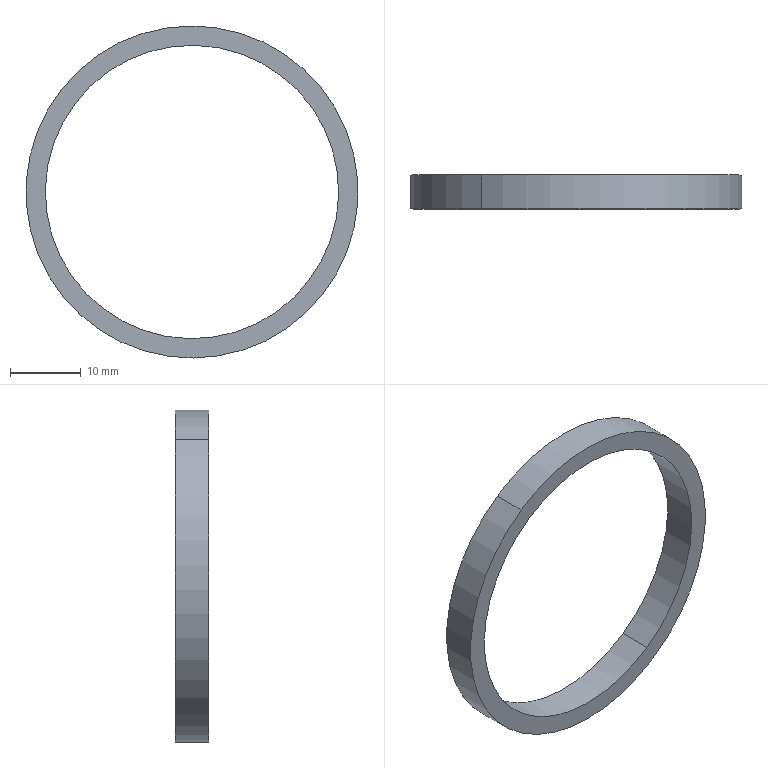Component | SolidWorks | 15-1 | 1 solid | 6 faces | box 47 x 4.8 x 47 mm | volume 1829 mm3 | cylinder 4 | plane 2 | commonest cylinder face diameters 41.52 x2 47 x2
build123d program:
from build123d import *

# Parameters (mm, degrees)
SKETCH1_R           = 23.5
SKETCH1_R_2         = 20.76
BOSS_EXTRUDE1_DEPTH = 4.8


with BuildPart() as part:
    # Sketch1 → Boss-Extrude1 (new body)
    with BuildSketch(Plane(origin=(0, 0, 0), x_dir=(1, 0, 0), z_dir=(0, 1, 0))):
        with Locations(Location((0, 0, 0), (0, 0, 270))):
            Circle(SKETCH1_R)
        with Locations(Location((0, 0, 0), (0, 0, 270))):
            Circle(SKETCH1_R_2, mode=Mode.SUBTRACT)
    extrude(amount=BOSS_EXTRUDE1_DEPTH)


solid = part.part

# Placed as in the assembly
solid = solid.moved(Location((0, -58.1, 0), (0, 0, 0)))
STEP:
#1=COLOUR_RGB('',0.7922,0.8196,0.9333);
#2=FILL_AREA_STYLE_COLOUR('',#1);
#3=FILL_AREA_STYLE('',(#2));
#4=SURFACE_STYLE_FILL_AREA(#3);
#5=SURFACE_SIDE_STYLE('',(#4));
#6=SURFACE_STYLE_USAGE(.BOTH.,#5);
#7=PRESENTATION_STYLE_ASSIGNMENT((#6));
#8=CARTESIAN_POINT('',(0.465,-2.098,-0.6722));
#9=VERTEX_POINT('',#8);
#10=CARTESIAN_POINT('',(-0.465,-2.098,0.6722));
#11=VERTEX_POINT('',#10);
#12=CARTESIAN_POINT('',(0.,-2.098,0.));
#13=DIRECTION('',(0.,1.,0.));
#14=DIRECTION('',(-0.5689,0.,0.8224));
#15=AXIS2_PLACEMENT_3D('',#12,#13,#14);
#16=CIRCLE('',#15,0.8173);
#17=EDGE_CURVE('',#9,#11,#16,.T.);
#18=ORIENTED_EDGE('',*,*,#17,.T.);
#19=CARTESIAN_POINT('',(-0.465,-2.287,0.6722));
#20=VERTEX_POINT('',#19);
#21=CARTESIAN_POINT('',(-0.465,-2.098,0.6722));
#22=DIRECTION('',(0.,-1.,0.));
#23=VECTOR('',#22,39.37);
#24=LINE('',#21,#23);
#25=EDGE_CURVE('',#11,#20,#24,.T.);
#26=ORIENTED_EDGE('',*,*,#25,.T.);
#27=CARTESIAN_POINT('',(0.465,-2.287,-0.6722));
#28=VERTEX_POINT('',#27);
#29=CARTESIAN_POINT('',(0.,-2.287,0.));
#30=DIRECTION('',(0.,1.,0.));
#31=DIRECTION('',(-0.5689,0.,0.8224));
#32=AXIS2_PLACEMENT_3D('',#29,#30,#31);
#33=CIRCLE('',#32,0.8173);
#34=EDGE_CURVE('',#28,#20,#33,.T.);
#35=ORIENTED_EDGE('',*,*,#34,.F.);
#36=CARTESIAN_POINT('',(0.465,-2.098,-0.6722));
#37=DIRECTION('',(0.,-1.,0.));
#38=VECTOR('',#37,39.37);
#39=LINE('',#36,#38);
#40=EDGE_CURVE('',#9,#28,#39,.T.);
#41=ORIENTED_EDGE('',*,*,#40,.F.);
#42=EDGE_LOOP('',(#18,#26,#35,#41));
#43=FACE_OUTER_BOUND('',#42,.T.);
#44=CARTESIAN_POINT('',(0.,-2.098,0.));
#45=DIRECTION('',(0.,-1.,0.));
#46=DIRECTION('',(0.5689,0.,-0.8224));
#47=AXIS2_PLACEMENT_3D('',#44,#45,#46);
#48=CYLINDRICAL_SURFACE('',#47,0.8173);
#49=ADVANCED_FACE('',(#43),#48,.F.);
#50=CARTESIAN_POINT('',(-0.5264,-2.098,0.7609));
#51=VERTEX_POINT('',#50);
#52=CARTESIAN_POINT('',(0.5264,-2.098,-0.7609));
#53=VERTEX_POINT('',#52);
#54=CARTESIAN_POINT('',(0.,-2.098,0.));
#55=DIRECTION('',(0.,1.,0.));
#56=DIRECTION('',(-0.5689,0.,0.8224));
#57=AXIS2_PLACEMENT_3D('',#54,#55,#56);
#58=CIRCLE('',#57,0.9252);
#59=EDGE_CURVE('',#51,#53,#58,.T.);
#60=ORIENTED_EDGE('',*,*,#59,.F.);
#61=CARTESIAN_POINT('',(-0.5264,-2.287,0.7609));
#62=VERTEX_POINT('',#61);
#63=CARTESIAN_POINT('',(-0.5264,-2.098,0.7609));
#64=DIRECTION('',(0.,-1.,0.));
#65=VECTOR('',#64,39.37);
#66=LINE('',#63,#65);
#67=EDGE_CURVE('',#51,#62,#66,.T.);
#68=ORIENTED_EDGE('',*,*,#67,.T.);
#69=CARTESIAN_POINT('',(0.5264,-2.287,-0.7609));
#70=VERTEX_POINT('',#69);
#71=CARTESIAN_POINT('',(0.,-2.287,0.));
#72=DIRECTION('',(0.,1.,0.));
#73=DIRECTION('',(-0.5689,0.,0.8224));
#74=AXIS2_PLACEMENT_3D('',#71,#72,#73);
#75=CIRCLE('',#74,0.9252);
#76=EDGE_CURVE('',#62,#70,#75,.T.);
#77=ORIENTED_EDGE('',*,*,#76,.T.);
#78=CARTESIAN_POINT('',(0.5264,-2.098,-0.7609));
#79=DIRECTION('',(0.,-1.,0.));
#80=VECTOR('',#79,39.37);
#81=LINE('',#78,#80);
#82=EDGE_CURVE('',#53,#70,#81,.T.);
#83=ORIENTED_EDGE('',*,*,#82,.F.);
#84=EDGE_LOOP('',(#60,#68,#77,#83));
#85=FACE_OUTER_BOUND('',#84,.T.);
#86=CARTESIAN_POINT('',(0.,-2.098,0.));
#87=DIRECTION('',(0.,-1.,0.));
#88=DIRECTION('',(0.5689,0.,-0.8224));
#89=AXIS2_PLACEMENT_3D('',#86,#87,#88);
#90=CYLINDRICAL_SURFACE('',#89,0.9252);
#91=ADVANCED_FACE('',(#85),#90,.T.);
#92=CARTESIAN_POINT('',(0.,-2.098,0.));
#93=DIRECTION('',(0.,1.,0.));
#94=DIRECTION('',(-0.5689,0.,0.8224));
#95=AXIS2_PLACEMENT_3D('',#92,#93,#94);
#96=CIRCLE('',#95,0.9252);
#97=EDGE_CURVE('',#53,#51,#96,.T.);
#98=ORIENTED_EDGE('',*,*,#97,.T.);
#99=ORIENTED_EDGE('',*,*,#59,.T.);
#100=EDGE_LOOP('',(#98,#99));
#101=FACE_OUTER_BOUND('',#100,.T.);
#102=ORIENTED_EDGE('',*,*,#17,.F.);
#103=CARTESIAN_POINT('',(0.,-2.098,0.));
#104=DIRECTION('',(0.,1.,0.));
#105=DIRECTION('',(-0.5689,0.,0.8224));
#106=AXIS2_PLACEMENT_3D('',#103,#104,#105);
#107=CIRCLE('',#106,0.8173);
#108=EDGE_CURVE('',#11,#9,#107,.T.);
#109=ORIENTED_EDGE('',*,*,#108,.F.);
#110=EDGE_LOOP('',(#102,#109));
#111=FACE_BOUND('',#110,.T.);
#112=CARTESIAN_POINT('',(0.,-2.098,0.));
#113=DIRECTION('',(0.,1.,0.));
#114=DIRECTION('',(-0.5689,0.,0.8224));
#115=AXIS2_PLACEMENT_3D('',#112,#113,#114);
#116=PLANE('',#115);
#117=ADVANCED_FACE('',(#101,#111),#116,.T.);
#118=CARTESIAN_POINT('',(0.,-2.287,0.));
#119=DIRECTION('',(0.,1.,0.));
#120=DIRECTION('',(-0.5689,0.,0.8224));
#121=AXIS2_PLACEMENT_3D('',#118,#119,#120);
#122=CIRCLE('',#121,0.9252);
#123=EDGE_CURVE('',#70,#62,#122,.T.);
#124=ORIENTED_EDGE('',*,*,#123,.F.);
#125=ORIENTED_EDGE('',*,*,#76,.F.);
#126=EDGE_LOOP('',(#124,#125));
#127=FACE_OUTER_BOUND('',#126,.T.);
#128=ORIENTED_EDGE('',*,*,#34,.T.);
#129=CARTESIAN_POINT('',(0.,-2.287,0.));
#130=DIRECTION('',(0.,1.,0.));
#131=DIRECTION('',(-0.5689,0.,0.8224));
#132=AXIS2_PLACEMENT_3D('',#129,#130,#131);
#133=CIRCLE('',#132,0.8173);
#134=EDGE_CURVE('',#20,#28,#133,.T.);
#135=ORIENTED_EDGE('',*,*,#134,.T.);
#136=EDGE_LOOP('',(#128,#135));
#137=FACE_BOUND('',#136,.T.);
#138=CARTESIAN_POINT('',(0.,-2.287,0.));
#139=DIRECTION('',(0.,1.,0.));
#140=DIRECTION('',(-0.5689,0.,0.8224));
#141=AXIS2_PLACEMENT_3D('',#138,#139,#140);
#142=PLANE('',#141);
#143=ADVANCED_FACE('',(#127,#137),#142,.F.);
#144=ORIENTED_EDGE('',*,*,#67,.F.);
#145=ORIENTED_EDGE('',*,*,#97,.F.);
#146=ORIENTED_EDGE('',*,*,#82,.T.);
#147=ORIENTED_EDGE('',*,*,#123,.T.);
#148=EDGE_LOOP('',(#144,#145,#146,#147));
#149=FACE_OUTER_BOUND('',#148,.T.);
#150=CARTESIAN_POINT('',(0.,-2.098,0.));
#151=DIRECTION('',(0.,-1.,0.));
#152=DIRECTION('',(0.5689,0.,-0.8224));
#153=AXIS2_PLACEMENT_3D('',#150,#151,#152);
#154=CYLINDRICAL_SURFACE('',#153,0.9252);
#155=ADVANCED_FACE('',(#149),#154,.T.);
#156=ORIENTED_EDGE('',*,*,#25,.F.);
#157=ORIENTED_EDGE('',*,*,#108,.T.);
#158=ORIENTED_EDGE('',*,*,#40,.T.);
#159=ORIENTED_EDGE('',*,*,#134,.F.);
#160=EDGE_LOOP('',(#156,#157,#158,#159));
#161=FACE_OUTER_BOUND('',#160,.T.);
#162=CARTESIAN_POINT('',(0.,-2.098,0.));
#163=DIRECTION('',(0.,-1.,0.));
#164=DIRECTION('',(0.5689,0.,-0.8224));
#165=AXIS2_PLACEMENT_3D('',#162,#163,#164);
#166=CYLINDRICAL_SURFACE('',#165,0.8173);
#167=ADVANCED_FACE('',(#161),#166,.F.);
#168=CLOSED_SHELL('',(#49,#91,#117,#143,#155,#167));
#169=MANIFOLD_SOLID_BREP('',#168);
#170=STYLED_ITEM('',(#7),#169);
#171=(LENGTH_UNIT()NAMED_UNIT(*)SI_UNIT($,.METRE.));
#172=LENGTH_MEASURE_WITH_UNIT(LENGTH_MEASURE(0.0254),#171);
#173=DIMENSIONAL_EXPONENTS(1.,0.,0.,0.,0.,0.,0.);
#174=(CONVERSION_BASED_UNIT('',#172)LENGTH_UNIT()NAMED_UNIT(#173));
#175=UNCERTAINTY_MEASURE_WITH_UNIT(LENGTH_MEASURE(0.00001),#174,'','');
#176=(NAMED_UNIT(*)PLANE_ANGLE_UNIT()SI_UNIT($,.RADIAN.));
#177=(NAMED_UNIT(*)SI_UNIT($,.STERADIAN.)SOLID_ANGLE_UNIT());
#178=(GEOMETRIC_REPRESENTATION_CONTEXT(3)GLOBAL_UNCERTAINTY_ASSIGNED_CONTEXT((#175))GLOBAL_UNIT_ASSIGNED_CONTEXT((#174,#176,#177))REPRESENTATION_CONTEXT('',''));
#179=MECHANICAL_DESIGN_GEOMETRIC_PRESENTATION_REPRESENTATION('',(#170),#178);
#180=PRESENTATION_LAYER_ASSIGNMENT('','',(#170));
#181=CARTESIAN_POINT('',(0.,0.,0.));
#182=DIRECTION('',(0.,0.,1.));
#183=DIRECTION('',(1.,0.,0.));
#184=AXIS2_PLACEMENT_3D('',#181,#182,#183);
#185=(LENGTH_UNIT()NAMED_UNIT(*)SI_UNIT($,.METRE.));
#186=LENGTH_MEASURE_WITH_UNIT(LENGTH_MEASURE(0.0254),#185);
#187=DIMENSIONAL_EXPONENTS(1.,0.,0.,0.,0.,0.,0.);
#188=(CONVERSION_BASED_UNIT('',#186)LENGTH_UNIT()NAMED_UNIT(#187));
#189=UNCERTAINTY_MEASURE_WITH_UNIT(LENGTH_MEASURE(0.00001),#188,'','');
#190=(NAMED_UNIT(*)PLANE_ANGLE_UNIT()SI_UNIT($,.RADIAN.));
#191=(NAMED_UNIT(*)SI_UNIT($,.STERADIAN.)SOLID_ANGLE_UNIT());
#192=(GEOMETRIC_REPRESENTATION_CONTEXT(3)GLOBAL_UNCERTAINTY_ASSIGNED_CONTEXT((#189))GLOBAL_UNIT_ASSIGNED_CONTEXT((#188,#190,#191))REPRESENTATION_CONTEXT('',''));
#193=ADVANCED_BREP_SHAPE_REPRESENTATION('',(#169,#184),#192);